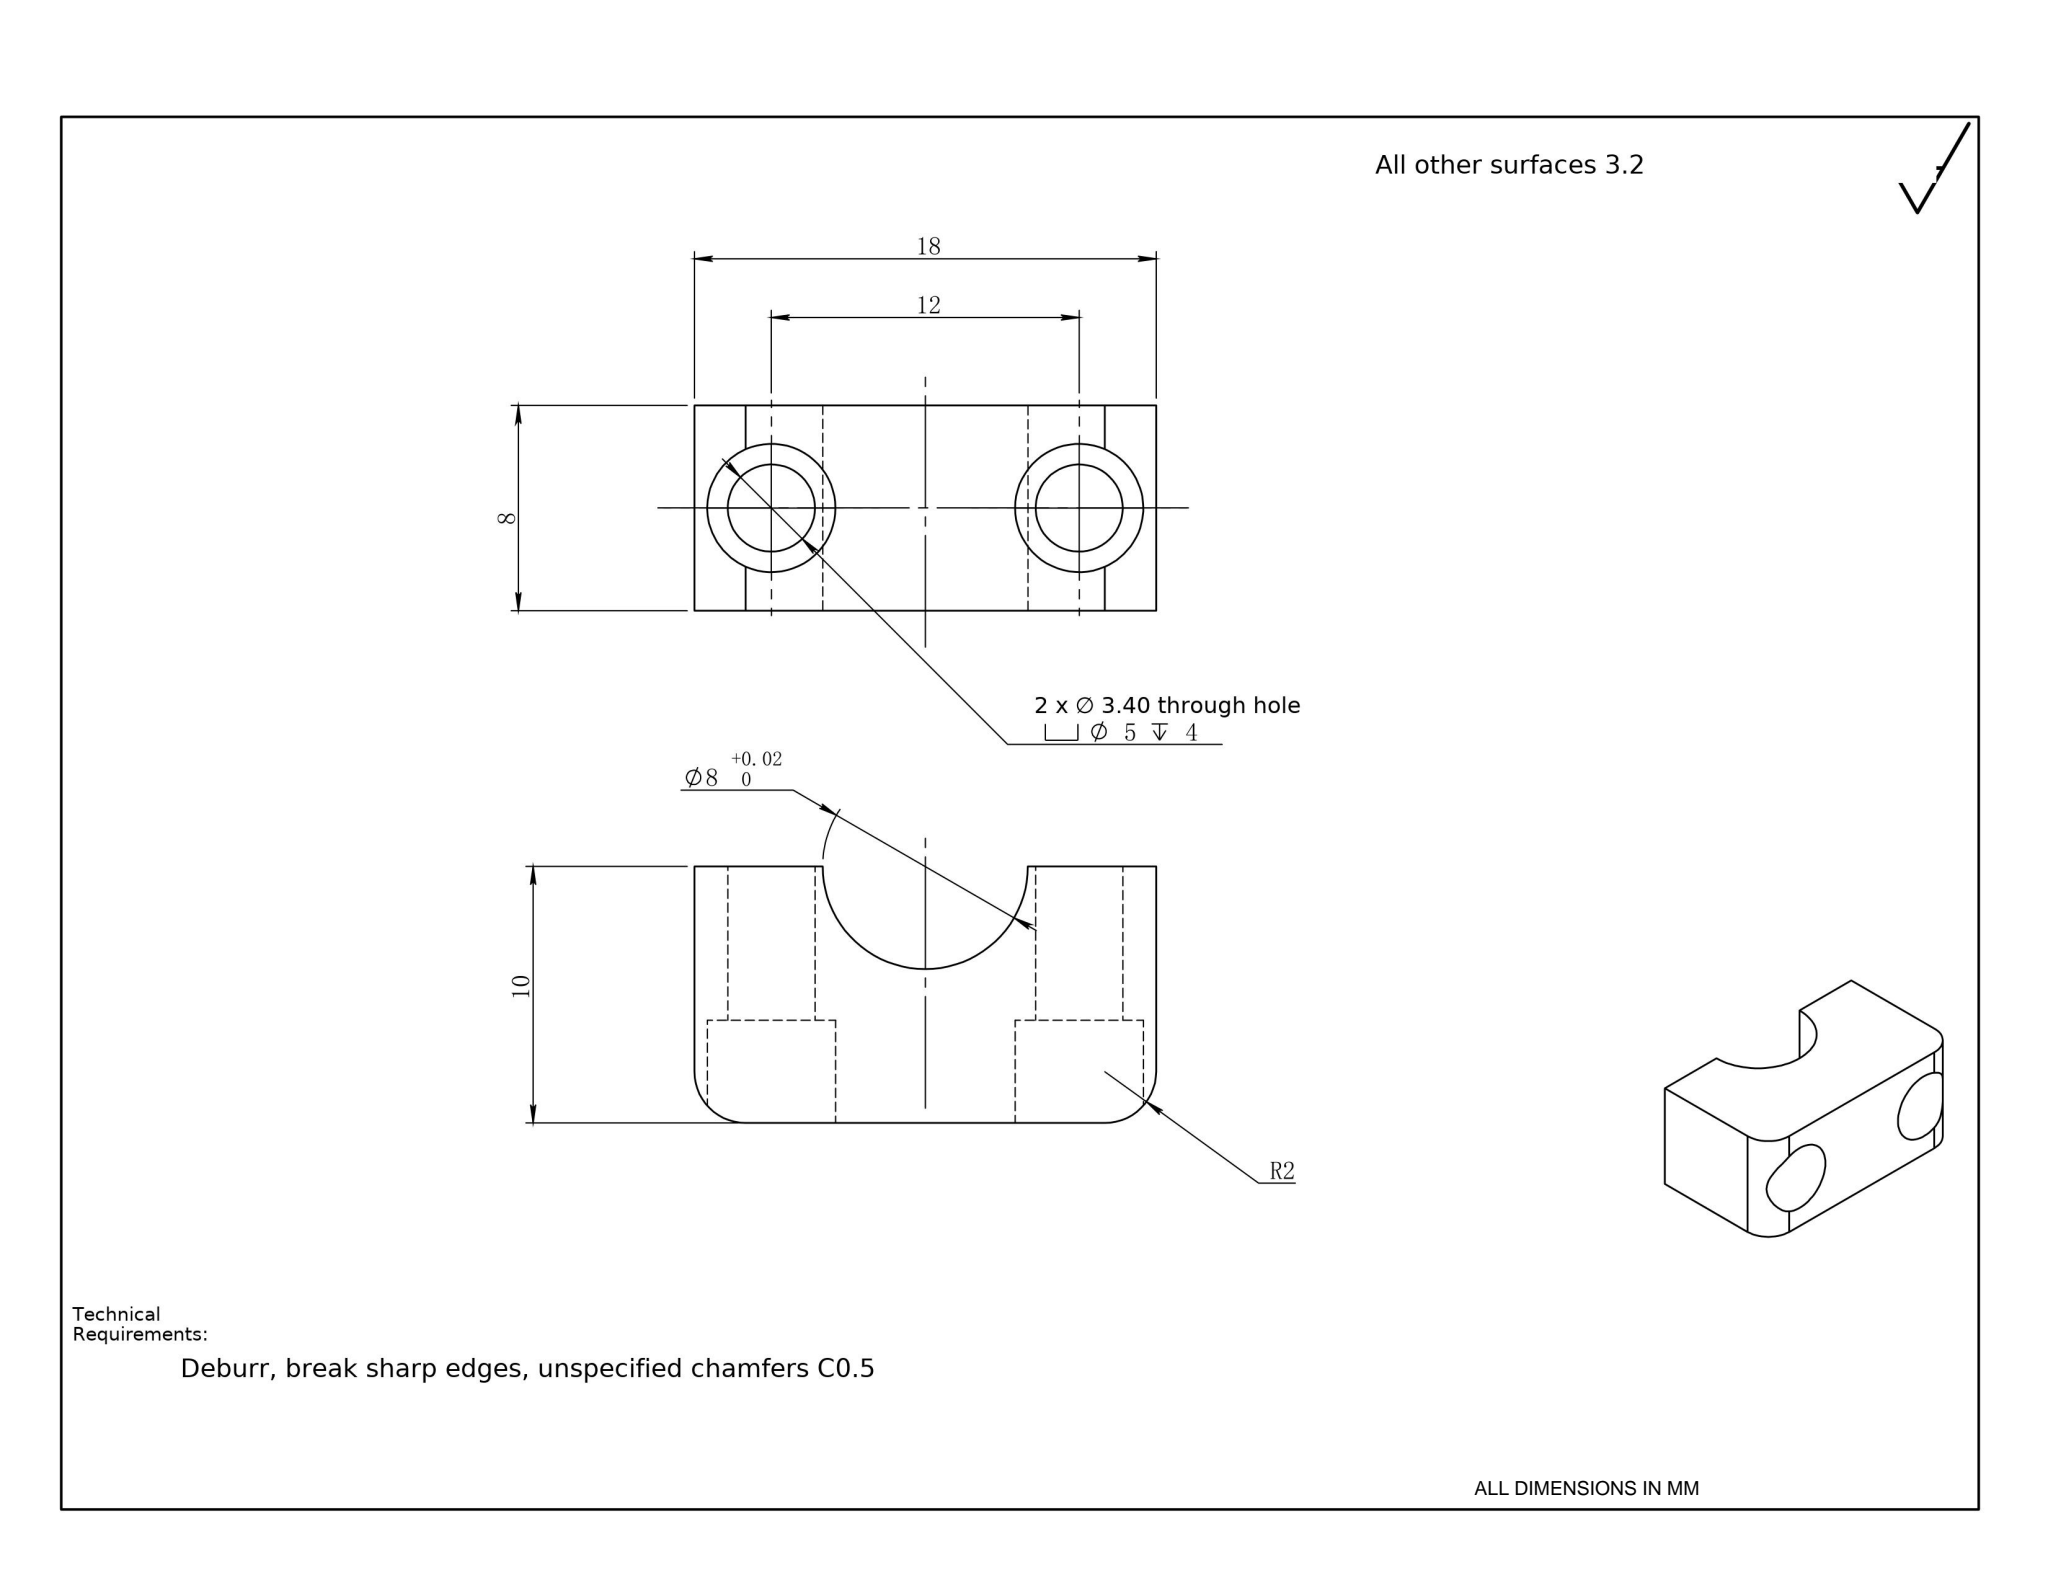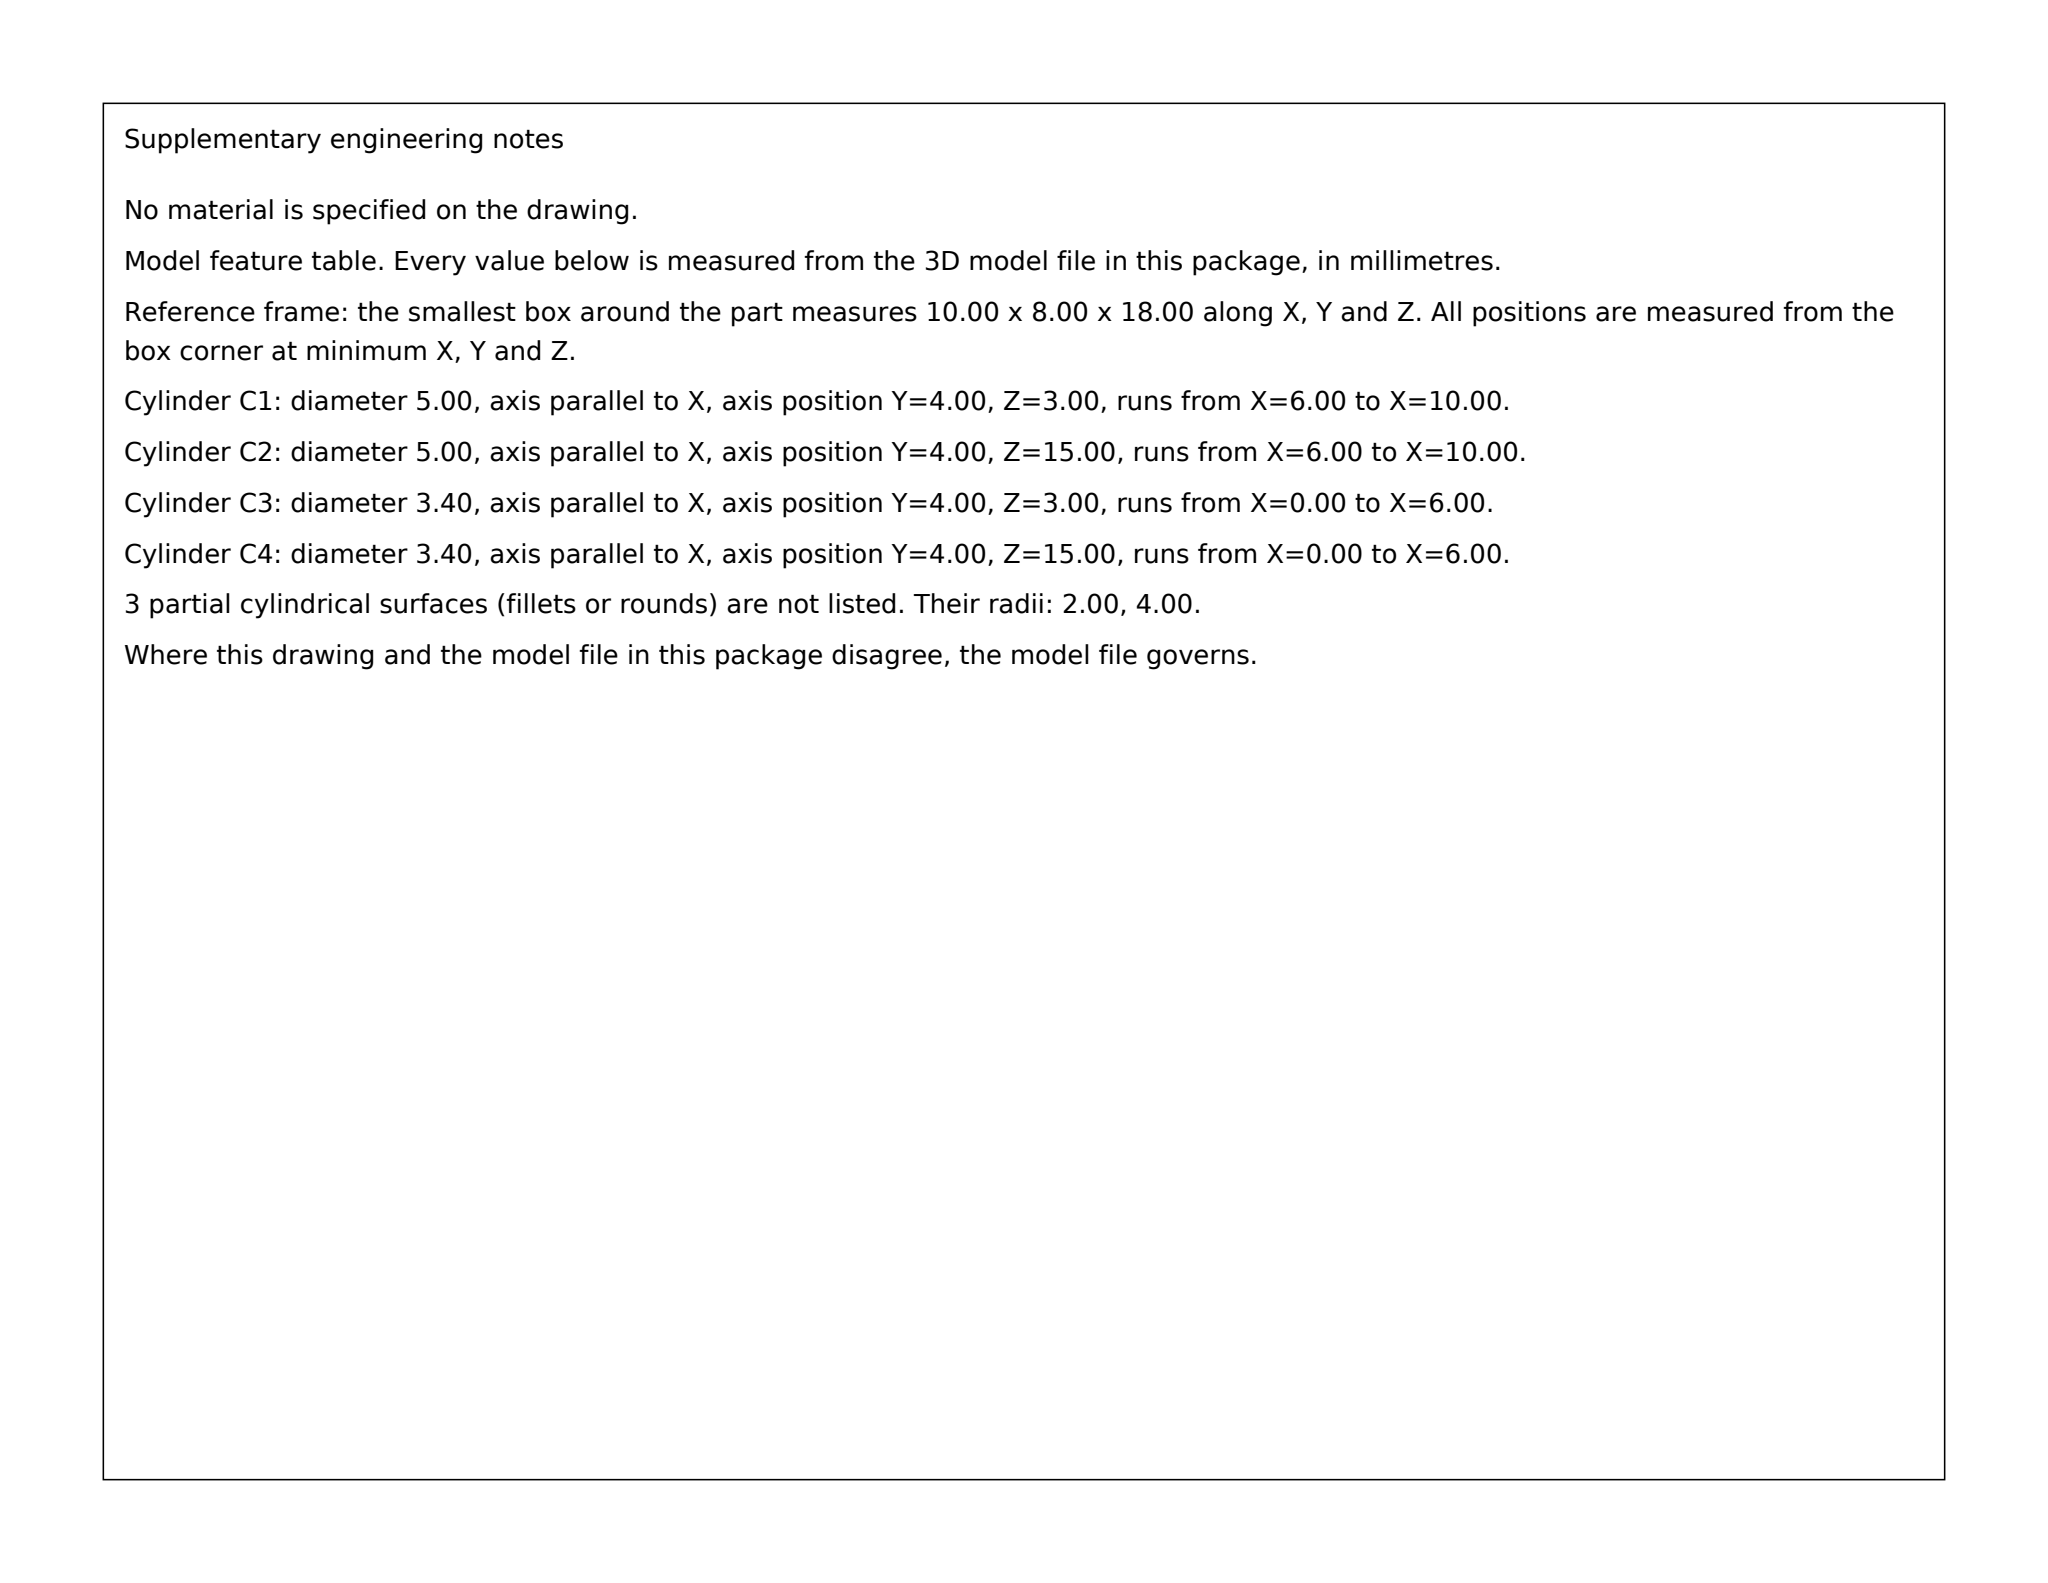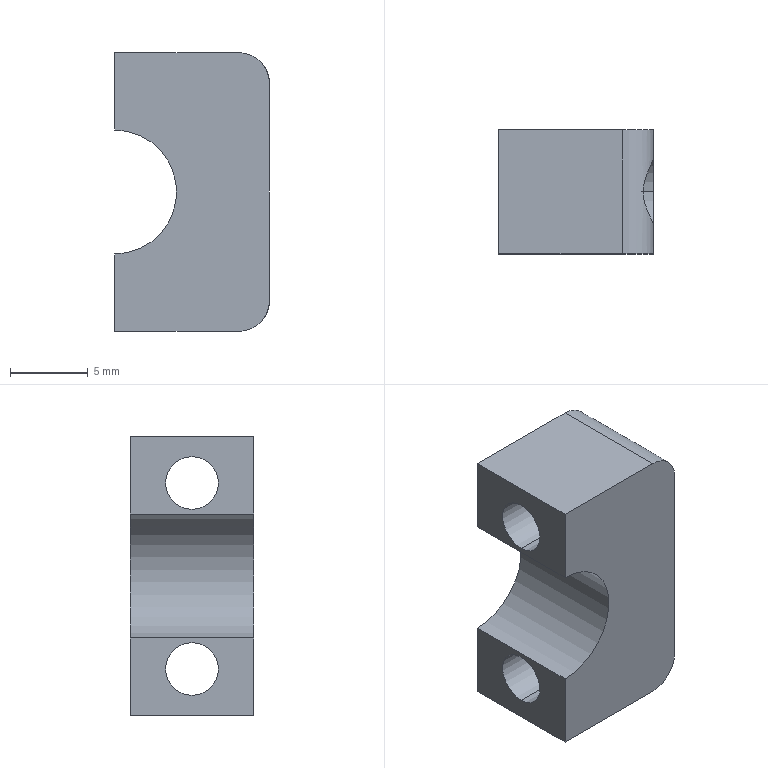Part | SolidWorks | mm | 1 solid | 20 faces | box 10 x 8 x 18 mm | volume 961 mm3 | cylinder 11 | plane 9 | commonest cylinder face diameters 5 x4 3.4 x4 4 x2 8 x1
STEP:
#1=CARTESIAN_POINT('',(1.,0.,8.5));
#2=VERTEX_POINT('',#1);
#3=CARTESIAN_POINT('',(1.,0.,3.5));
#4=VERTEX_POINT('',#3);
#5=CARTESIAN_POINT('',(1.,0.,6.));
#6=DIRECTION('',(1.,0.,0.));
#7=DIRECTION('',(0.,0.,-1.));
#8=AXIS2_PLACEMENT_3D('',#5,#6,#7);
#9=CIRCLE('',#8,2.5);
#10=EDGE_CURVE('',#2,#4,#9,.T.);
#11=ORIENTED_EDGE('',*,*,#10,.F.);
#12=CARTESIAN_POINT('',(4.323,0.,8.5));
#13=VERTEX_POINT('',#12);
#14=CARTESIAN_POINT('',(5.,0.,8.5));
#15=DIRECTION('',(1.,0.,0.));
#16=VECTOR('',#15,1000.);
#17=LINE('',#14,#16);
#18=EDGE_CURVE('',#2,#13,#17,.T.);
#19=ORIENTED_EDGE('',*,*,#18,.T.);
#20=CARTESIAN_POINT('',(5.,-2.291,7.));
#21=VERTEX_POINT('',#20);
#22=CARTESIAN_POINT('',(4.323,0.,8.5));
#23=CARTESIAN_POINT('',(4.323,-0.126,8.5));
#24=CARTESIAN_POINT('',(4.334,-0.2501,8.49));
#25=CARTESIAN_POINT('',(4.374,-0.4931,8.454));
#26=CARTESIAN_POINT('',(4.403,-0.6133,8.427));
#27=CARTESIAN_POINT('',(4.504,-0.958,8.322));
#28=CARTESIAN_POINT('',(4.591,-1.17,8.222));
#29=CARTESIAN_POINT('',(4.759,-1.565,7.964));
#30=CARTESIAN_POINT('',(4.839,-1.742,7.81));
#31=CARTESIAN_POINT('',(4.961,-2.058,7.44));
#32=CARTESIAN_POINT('',(5.,-2.19,7.231));
#33=CARTESIAN_POINT('',(5.,-2.291,7.));
#34=B_SPLINE_CURVE_WITH_KNOTS('',3,(#22,#23,#24,#25,#26,#27,#28,#29,#30,#31,#32,#33),.UNSPECIFIED.,.F.,.F.,(4,2,2,2,2,4),(0.002976,0.003348,0.00372,0.004464,0.005207,0.005951),.UNSPECIFIED.);
#35=EDGE_CURVE('',#13,#21,#34,.T.);
#36=ORIENTED_EDGE('',*,*,#35,.T.);
#37=CARTESIAN_POINT('',(5.,0.,3.5));
#38=VERTEX_POINT('',#37);
#39=CARTESIAN_POINT('',(5.,0.,6.));
#40=DIRECTION('',(1.,0.,0.));
#41=DIRECTION('',(0.,0.,-1.));
#42=AXIS2_PLACEMENT_3D('',#39,#40,#41);
#43=CIRCLE('',#42,2.5);
#44=EDGE_CURVE('',#21,#38,#43,.T.);
#45=ORIENTED_EDGE('',*,*,#44,.T.);
#46=CARTESIAN_POINT('',(5.,0.,3.5));
#47=DIRECTION('',(1.,0.,0.));
#48=VECTOR('',#47,1000.);
#49=LINE('',#46,#48);
#50=EDGE_CURVE('',#4,#38,#49,.T.);
#51=ORIENTED_EDGE('',*,*,#50,.F.);
#52=EDGE_LOOP('',(#11,#19,#36,#45,#51));
#53=FACE_OUTER_BOUND('',#52,.T.);
#54=CARTESIAN_POINT('',(5.,0.,6.));
#55=DIRECTION('',(1.,0.,0.));
#56=DIRECTION('',(0.,0.,-1.));
#57=AXIS2_PLACEMENT_3D('',#54,#55,#56);
#58=CYLINDRICAL_SURFACE('',#57,2.5);
#59=ADVANCED_FACE('',(#53),#58,.F.);
#60=CARTESIAN_POINT('',(-5.,0.,7.7));
#61=VERTEX_POINT('',#60);
#62=CARTESIAN_POINT('',(-5.,0.,4.3));
#63=VERTEX_POINT('',#62);
#64=CARTESIAN_POINT('',(-5.,0.,6.));
#65=DIRECTION('',(1.,0.,0.));
#66=DIRECTION('',(0.,0.,-1.));
#67=AXIS2_PLACEMENT_3D('',#64,#65,#66);
#68=CIRCLE('',#67,1.7);
#69=EDGE_CURVE('',#61,#63,#68,.T.);
#70=ORIENTED_EDGE('',*,*,#69,.F.);
#71=CARTESIAN_POINT('',(1.,0.,7.7));
#72=VERTEX_POINT('',#71);
#73=CARTESIAN_POINT('',(5.,0.,7.7));
#74=DIRECTION('',(1.,0.,0.));
#75=VECTOR('',#74,1000.);
#76=LINE('',#73,#75);
#77=EDGE_CURVE('',#61,#72,#76,.T.);
#78=ORIENTED_EDGE('',*,*,#77,.T.);
#79=CARTESIAN_POINT('',(1.,0.,4.3));
#80=VERTEX_POINT('',#79);
#81=CARTESIAN_POINT('',(1.,0.,6.));
#82=DIRECTION('',(1.,0.,0.));
#83=DIRECTION('',(0.,0.,-1.));
#84=AXIS2_PLACEMENT_3D('',#81,#82,#83);
#85=CIRCLE('',#84,1.7);
#86=EDGE_CURVE('',#72,#80,#85,.T.);
#87=ORIENTED_EDGE('',*,*,#86,.T.);
#88=CARTESIAN_POINT('',(5.,0.,4.3));
#89=DIRECTION('',(1.,0.,0.));
#90=VECTOR('',#89,1000.);
#91=LINE('',#88,#90);
#92=EDGE_CURVE('',#63,#80,#91,.T.);
#93=ORIENTED_EDGE('',*,*,#92,.F.);
#94=EDGE_LOOP('',(#70,#78,#87,#93));
#95=FACE_OUTER_BOUND('',#94,.T.);
#96=CARTESIAN_POINT('',(5.,0.,6.));
#97=DIRECTION('',(1.,0.,0.));
#98=DIRECTION('',(0.,0.,-1.));
#99=AXIS2_PLACEMENT_3D('',#96,#97,#98);
#100=CYLINDRICAL_SURFACE('',#99,1.7);
#101=ADVANCED_FACE('',(#95),#100,.F.);
#102=CARTESIAN_POINT('',(1.,0.,-3.5));
#103=VERTEX_POINT('',#102);
#104=CARTESIAN_POINT('',(1.,0.,-8.5));
#105=VERTEX_POINT('',#104);
#106=CARTESIAN_POINT('',(1.,0.,-6.));
#107=DIRECTION('',(1.,0.,0.));
#108=DIRECTION('',(0.,0.,-1.));
#109=AXIS2_PLACEMENT_3D('',#106,#107,#108);
#110=CIRCLE('',#109,2.5);
#111=EDGE_CURVE('',#103,#105,#110,.T.);
#112=ORIENTED_EDGE('',*,*,#111,.F.);
#113=CARTESIAN_POINT('',(5.,0.,-3.5));
#114=VERTEX_POINT('',#113);
#115=CARTESIAN_POINT('',(5.,0.,-3.5));
#116=DIRECTION('',(1.,0.,0.));
#117=VECTOR('',#116,1000.);
#118=LINE('',#115,#117);
#119=EDGE_CURVE('',#103,#114,#118,.T.);
#120=ORIENTED_EDGE('',*,*,#119,.T.);
#121=CARTESIAN_POINT('',(5.,-2.291,-7.));
#122=VERTEX_POINT('',#121);
#123=CARTESIAN_POINT('',(5.,0.,-6.));
#124=DIRECTION('',(1.,0.,0.));
#125=DIRECTION('',(0.,0.,-1.));
#126=AXIS2_PLACEMENT_3D('',#123,#124,#125);
#127=CIRCLE('',#126,2.5);
#128=EDGE_CURVE('',#114,#122,#127,.T.);
#129=ORIENTED_EDGE('',*,*,#128,.T.);
#130=CARTESIAN_POINT('',(4.323,-0.,-8.5));
#131=VERTEX_POINT('',#130);
#132=CARTESIAN_POINT('',(5.,-2.291,-7.));
#133=CARTESIAN_POINT('',(5.,-2.19,-7.231));
#134=CARTESIAN_POINT('',(4.961,-2.058,-7.44));
#135=CARTESIAN_POINT('',(4.839,-1.742,-7.81));
#136=CARTESIAN_POINT('',(4.759,-1.565,-7.964));
#137=CARTESIAN_POINT('',(4.591,-1.17,-8.222));
#138=CARTESIAN_POINT('',(4.504,-0.9577,-8.322));
#139=CARTESIAN_POINT('',(4.403,-0.6135,-8.427));
#140=CARTESIAN_POINT('',(4.374,-0.493,-8.454));
#141=CARTESIAN_POINT('',(4.334,-0.2498,-8.491));
#142=CARTESIAN_POINT('',(4.323,-0.1261,-8.5));
#143=CARTESIAN_POINT('',(4.323,-0.,-8.5));
#144=B_SPLINE_CURVE_WITH_KNOTS('',3,(#132,#133,#134,#135,#136,#137,#138,#139,#140,#141,#142,#143),.UNSPECIFIED.,.F.,.F.,(4,2,2,2,2,4),(0.,0.0007441,0.001488,0.002232,0.002604,0.002976),.UNSPECIFIED.);
#145=EDGE_CURVE('',#122,#131,#144,.T.);
#146=ORIENTED_EDGE('',*,*,#145,.T.);
#147=CARTESIAN_POINT('',(5.,0.,-8.5));
#148=DIRECTION('',(1.,0.,0.));
#149=VECTOR('',#148,1000.);
#150=LINE('',#147,#149);
#151=EDGE_CURVE('',#105,#131,#150,.T.);
#152=ORIENTED_EDGE('',*,*,#151,.F.);
#153=EDGE_LOOP('',(#112,#120,#129,#146,#152));
#154=FACE_OUTER_BOUND('',#153,.T.);
#155=CARTESIAN_POINT('',(5.,0.,-6.));
#156=DIRECTION('',(1.,0.,0.));
#157=DIRECTION('',(0.,0.,-1.));
#158=AXIS2_PLACEMENT_3D('',#155,#156,#157);
#159=CYLINDRICAL_SURFACE('',#158,2.5);
#160=ADVANCED_FACE('',(#154),#159,.F.);
#161=CARTESIAN_POINT('',(-5.,0.,-4.3));
#162=VERTEX_POINT('',#161);
#163=CARTESIAN_POINT('',(-5.,0.,-7.7));
#164=VERTEX_POINT('',#163);
#165=CARTESIAN_POINT('',(-5.,0.,-6.));
#166=DIRECTION('',(1.,0.,0.));
#167=DIRECTION('',(0.,0.,-1.));
#168=AXIS2_PLACEMENT_3D('',#165,#166,#167);
#169=CIRCLE('',#168,1.7);
#170=EDGE_CURVE('',#162,#164,#169,.T.);
#171=ORIENTED_EDGE('',*,*,#170,.F.);
#172=CARTESIAN_POINT('',(1.,0.,-4.3));
#173=VERTEX_POINT('',#172);
#174=CARTESIAN_POINT('',(5.,0.,-4.3));
#175=DIRECTION('',(1.,0.,0.));
#176=VECTOR('',#175,1000.);
#177=LINE('',#174,#176);
#178=EDGE_CURVE('',#162,#173,#177,.T.);
#179=ORIENTED_EDGE('',*,*,#178,.T.);
#180=CARTESIAN_POINT('',(1.,0.,-7.7));
#181=VERTEX_POINT('',#180);
#182=CARTESIAN_POINT('',(1.,0.,-6.));
#183=DIRECTION('',(1.,0.,0.));
#184=DIRECTION('',(0.,0.,-1.));
#185=AXIS2_PLACEMENT_3D('',#182,#183,#184);
#186=CIRCLE('',#185,1.7);
#187=EDGE_CURVE('',#173,#181,#186,.T.);
#188=ORIENTED_EDGE('',*,*,#187,.T.);
#189=CARTESIAN_POINT('',(5.,0.,-7.7));
#190=DIRECTION('',(1.,0.,0.));
#191=VECTOR('',#190,1000.);
#192=LINE('',#189,#191);
#193=EDGE_CURVE('',#164,#181,#192,.T.);
#194=ORIENTED_EDGE('',*,*,#193,.F.);
#195=EDGE_LOOP('',(#171,#179,#188,#194));
#196=FACE_OUTER_BOUND('',#195,.T.);
#197=CARTESIAN_POINT('',(5.,0.,-6.));
#198=DIRECTION('',(1.,0.,0.));
#199=DIRECTION('',(0.,0.,-1.));
#200=AXIS2_PLACEMENT_3D('',#197,#198,#199);
#201=CYLINDRICAL_SURFACE('',#200,1.7);
#202=ADVANCED_FACE('',(#196),#201,.F.);
#203=CARTESIAN_POINT('',(-5.,0.,-6.));
#204=DIRECTION('',(1.,0.,0.));
#205=DIRECTION('',(0.,0.,-1.));
#206=AXIS2_PLACEMENT_3D('',#203,#204,#205);
#207=CIRCLE('',#206,1.7);
#208=EDGE_CURVE('',#164,#162,#207,.T.);
#209=ORIENTED_EDGE('',*,*,#208,.T.);
#210=ORIENTED_EDGE('',*,*,#170,.T.);
#211=EDGE_LOOP('',(#209,#210));
#212=FACE_BOUND('',#211,.T.);
#213=CARTESIAN_POINT('',(-5.,-4.,-9.));
#214=VERTEX_POINT('',#213);
#215=CARTESIAN_POINT('',(-5.,-4.,-4.));
#216=VERTEX_POINT('',#215);
#217=CARTESIAN_POINT('',(-5.,-4.,9.));
#218=DIRECTION('',(0.,0.,1.));
#219=VECTOR('',#218,1000.);
#220=LINE('',#217,#219);
#221=EDGE_CURVE('',#214,#216,#220,.T.);
#222=ORIENTED_EDGE('',*,*,#221,.T.);
#223=CARTESIAN_POINT('',(-5.,4.,-4.));
#224=VERTEX_POINT('',#223);
#225=CARTESIAN_POINT('',(-5.,-4.,-4.));
#226=DIRECTION('',(0.,1.,0.));
#227=VECTOR('',#226,1000.);
#228=LINE('',#225,#227);
#229=EDGE_CURVE('',#216,#224,#228,.T.);
#230=ORIENTED_EDGE('',*,*,#229,.T.);
#231=CARTESIAN_POINT('',(-5.,4.,-9.));
#232=VERTEX_POINT('',#231);
#233=CARTESIAN_POINT('',(-5.,4.,9.));
#234=DIRECTION('',(0.,0.,1.));
#235=VECTOR('',#234,1000.);
#236=LINE('',#233,#235);
#237=EDGE_CURVE('',#232,#224,#236,.T.);
#238=ORIENTED_EDGE('',*,*,#237,.F.);
#239=CARTESIAN_POINT('',(-5.,4.,-9.));
#240=DIRECTION('',(0.,-1.,0.));
#241=VECTOR('',#240,1000.);
#242=LINE('',#239,#241);
#243=EDGE_CURVE('',#232,#214,#242,.T.);
#244=ORIENTED_EDGE('',*,*,#243,.T.);
#245=EDGE_LOOP('',(#222,#230,#238,#244));
#246=FACE_OUTER_BOUND('',#245,.T.);
#247=CARTESIAN_POINT('',(-5.,4.,9.));
#248=DIRECTION('',(1.,0.,0.));
#249=DIRECTION('',(0.,0.,-1.));
#250=AXIS2_PLACEMENT_3D('',#247,#248,#249);
#251=PLANE('',#250);
#252=ADVANCED_FACE('',(#212,#246),#251,.F.);
#253=CARTESIAN_POINT('',(5.,-4.,7.));
#254=VERTEX_POINT('',#253);
#255=CARTESIAN_POINT('',(5.,-4.,-7.));
#256=VERTEX_POINT('',#255);
#257=CARTESIAN_POINT('',(5.,-4.,9.));
#258=DIRECTION('',(0.,0.,-1.));
#259=VECTOR('',#258,1000.);
#260=LINE('',#257,#259);
#261=EDGE_CURVE('',#254,#256,#260,.T.);
#262=ORIENTED_EDGE('',*,*,#261,.T.);
#263=CARTESIAN_POINT('',(5.,4.,-7.));
#264=DIRECTION('',(0.,1.,0.));
#265=VECTOR('',#264,1000.);
#266=LINE('',#263,#265);
#267=EDGE_CURVE('',#256,#122,#266,.T.);
#268=ORIENTED_EDGE('',*,*,#267,.T.);
#269=ORIENTED_EDGE('',*,*,#128,.F.);
#270=CARTESIAN_POINT('',(5.,2.291,-7.));
#271=VERTEX_POINT('',#270);
#272=CARTESIAN_POINT('',(5.,0.,-6.));
#273=DIRECTION('',(1.,0.,0.));
#274=DIRECTION('',(0.,0.,-1.));
#275=AXIS2_PLACEMENT_3D('',#272,#273,#274);
#276=CIRCLE('',#275,2.5);
#277=EDGE_CURVE('',#271,#114,#276,.T.);
#278=ORIENTED_EDGE('',*,*,#277,.F.);
#279=CARTESIAN_POINT('',(5.,4.,-7.));
#280=VERTEX_POINT('',#279);
#281=CARTESIAN_POINT('',(5.,4.,-7.));
#282=DIRECTION('',(0.,1.,0.));
#283=VECTOR('',#282,1000.);
#284=LINE('',#281,#283);
#285=EDGE_CURVE('',#271,#280,#284,.T.);
#286=ORIENTED_EDGE('',*,*,#285,.T.);
#287=CARTESIAN_POINT('',(5.,4.,7.));
#288=VERTEX_POINT('',#287);
#289=CARTESIAN_POINT('',(5.,4.,9.));
#290=DIRECTION('',(0.,0.,-1.));
#291=VECTOR('',#290,1000.);
#292=LINE('',#289,#291);
#293=EDGE_CURVE('',#288,#280,#292,.T.);
#294=ORIENTED_EDGE('',*,*,#293,.F.);
#295=CARTESIAN_POINT('',(5.,2.291,7.));
#296=VERTEX_POINT('',#295);
#297=CARTESIAN_POINT('',(5.,4.,7.));
#298=DIRECTION('',(0.,-1.,0.));
#299=VECTOR('',#298,1000.);
#300=LINE('',#297,#299);
#301=EDGE_CURVE('',#288,#296,#300,.T.);
#302=ORIENTED_EDGE('',*,*,#301,.T.);
#303=CARTESIAN_POINT('',(5.,0.,6.));
#304=DIRECTION('',(1.,0.,0.));
#305=DIRECTION('',(0.,0.,-1.));
#306=AXIS2_PLACEMENT_3D('',#303,#304,#305);
#307=CIRCLE('',#306,2.5);
#308=EDGE_CURVE('',#38,#296,#307,.T.);
#309=ORIENTED_EDGE('',*,*,#308,.F.);
#310=ORIENTED_EDGE('',*,*,#44,.F.);
#311=CARTESIAN_POINT('',(5.,4.,7.));
#312=DIRECTION('',(0.,-1.,0.));
#313=VECTOR('',#312,1000.);
#314=LINE('',#311,#313);
#315=EDGE_CURVE('',#21,#254,#314,.T.);
#316=ORIENTED_EDGE('',*,*,#315,.T.);
#317=EDGE_LOOP('',(#262,#268,#269,#278,#286,#294,#302,#309,#310,#316));
#318=FACE_OUTER_BOUND('',#317,.T.);
#319=CARTESIAN_POINT('',(5.,4.,9.));
#320=DIRECTION('',(-1.,0.,0.));
#321=DIRECTION('',(0.,0.,1.));
#322=AXIS2_PLACEMENT_3D('',#319,#320,#321);
#323=PLANE('',#322);
#324=ADVANCED_FACE('',(#318),#323,.F.);
#325=CARTESIAN_POINT('',(3.,4.,-9.));
#326=VERTEX_POINT('',#325);
#327=CARTESIAN_POINT('',(-5.,4.,-9.));
#328=DIRECTION('',(-1.,0.,0.));
#329=VECTOR('',#328,1000.);
#330=LINE('',#327,#329);
#331=EDGE_CURVE('',#326,#232,#330,.T.);
#332=ORIENTED_EDGE('',*,*,#331,.F.);
#333=CARTESIAN_POINT('',(3.,-4.,-9.));
#334=VERTEX_POINT('',#333);
#335=CARTESIAN_POINT('',(3.,4.,-9.));
#336=DIRECTION('',(0.,-1.,0.));
#337=VECTOR('',#336,1000.);
#338=LINE('',#335,#337);
#339=EDGE_CURVE('',#326,#334,#338,.T.);
#340=ORIENTED_EDGE('',*,*,#339,.T.);
#341=CARTESIAN_POINT('',(-5.,-4.,-9.));
#342=DIRECTION('',(-1.,0.,0.));
#343=VECTOR('',#342,1000.);
#344=LINE('',#341,#343);
#345=EDGE_CURVE('',#334,#214,#344,.T.);
#346=ORIENTED_EDGE('',*,*,#345,.T.);
#347=ORIENTED_EDGE('',*,*,#243,.F.);
#348=EDGE_LOOP('',(#332,#340,#346,#347));
#349=FACE_OUTER_BOUND('',#348,.T.);
#350=CARTESIAN_POINT('',(-5.,4.,-9.));
#351=DIRECTION('',(0.,0.,1.));
#352=DIRECTION('',(1.,0.,0.));
#353=AXIS2_PLACEMENT_3D('',#350,#351,#352);
#354=PLANE('',#353);
#355=ADVANCED_FACE('',(#349),#354,.F.);
#356=CARTESIAN_POINT('',(-5.,0.,6.));
#357=DIRECTION('',(1.,0.,0.));
#358=DIRECTION('',(0.,0.,-1.));
#359=AXIS2_PLACEMENT_3D('',#356,#357,#358);
#360=CIRCLE('',#359,1.7);
#361=EDGE_CURVE('',#63,#61,#360,.T.);
#362=ORIENTED_EDGE('',*,*,#361,.T.);
#363=ORIENTED_EDGE('',*,*,#69,.T.);
#364=EDGE_LOOP('',(#362,#363));
#365=FACE_BOUND('',#364,.T.);
#366=CARTESIAN_POINT('',(-5.,4.,4.));
#367=VERTEX_POINT('',#366);
#368=CARTESIAN_POINT('',(-5.,4.,9.));
#369=VERTEX_POINT('',#368);
#370=CARTESIAN_POINT('',(-5.,4.,9.));
#371=DIRECTION('',(0.,0.,1.));
#372=VECTOR('',#371,1000.);
#373=LINE('',#370,#372);
#374=EDGE_CURVE('',#367,#369,#373,.T.);
#375=ORIENTED_EDGE('',*,*,#374,.F.);
#376=CARTESIAN_POINT('',(-5.,-4.,4.));
#377=VERTEX_POINT('',#376);
#378=CARTESIAN_POINT('',(-5.,-4.,4.));
#379=DIRECTION('',(0.,-1.,0.));
#380=VECTOR('',#379,1000.);
#381=LINE('',#378,#380);
#382=EDGE_CURVE('',#367,#377,#381,.T.);
#383=ORIENTED_EDGE('',*,*,#382,.T.);
#384=CARTESIAN_POINT('',(-5.,-4.,9.));
#385=VERTEX_POINT('',#384);
#386=CARTESIAN_POINT('',(-5.,-4.,9.));
#387=DIRECTION('',(0.,0.,1.));
#388=VECTOR('',#387,1000.);
#389=LINE('',#386,#388);
#390=EDGE_CURVE('',#377,#385,#389,.T.);
#391=ORIENTED_EDGE('',*,*,#390,.T.);
#392=CARTESIAN_POINT('',(-5.,4.,9.));
#393=DIRECTION('',(0.,-1.,0.));
#394=VECTOR('',#393,1000.);
#395=LINE('',#392,#394);
#396=EDGE_CURVE('',#369,#385,#395,.T.);
#397=ORIENTED_EDGE('',*,*,#396,.F.);
#398=EDGE_LOOP('',(#375,#383,#391,#397));
#399=FACE_OUTER_BOUND('',#398,.T.);
#400=CARTESIAN_POINT('',(-5.,4.,9.));
#401=DIRECTION('',(1.,0.,0.));
#402=DIRECTION('',(0.,0.,-1.));
#403=AXIS2_PLACEMENT_3D('',#400,#401,#402);
#404=PLANE('',#403);
#405=ADVANCED_FACE('',(#365,#399),#404,.F.);
#406=CARTESIAN_POINT('',(3.,-4.,9.));
#407=VERTEX_POINT('',#406);
#408=CARTESIAN_POINT('',(-5.,-4.,9.));
#409=DIRECTION('',(1.,0.,0.));
#410=VECTOR('',#409,1000.);
#411=LINE('',#408,#410);
#412=EDGE_CURVE('',#385,#407,#411,.T.);
#413=ORIENTED_EDGE('',*,*,#412,.T.);
#414=CARTESIAN_POINT('',(3.,4.,9.));
#415=VERTEX_POINT('',#414);
#416=CARTESIAN_POINT('',(3.,4.,9.));
#417=DIRECTION('',(0.,1.,0.));
#418=VECTOR('',#417,1000.);
#419=LINE('',#416,#418);
#420=EDGE_CURVE('',#407,#415,#419,.T.);
#421=ORIENTED_EDGE('',*,*,#420,.T.);
#422=CARTESIAN_POINT('',(-5.,4.,9.));
#423=DIRECTION('',(1.,0.,0.));
#424=VECTOR('',#423,1000.);
#425=LINE('',#422,#424);
#426=EDGE_CURVE('',#369,#415,#425,.T.);
#427=ORIENTED_EDGE('',*,*,#426,.F.);
#428=ORIENTED_EDGE('',*,*,#396,.T.);
#429=EDGE_LOOP('',(#413,#421,#427,#428));
#430=FACE_OUTER_BOUND('',#429,.T.);
#431=CARTESIAN_POINT('',(-5.,4.,9.));
#432=DIRECTION('',(0.,0.,-1.));
#433=DIRECTION('',(-1.,0.,0.));
#434=AXIS2_PLACEMENT_3D('',#431,#432,#433);
#435=PLANE('',#434);
#436=ADVANCED_FACE('',(#430),#435,.F.);
#437=ORIENTED_EDGE('',*,*,#293,.T.);
#438=CARTESIAN_POINT('',(3.,4.,-7.));
#439=DIRECTION('',(0.,1.,0.));
#440=DIRECTION('',(0.,0.,-1.));
#441=AXIS2_PLACEMENT_3D('',#438,#439,#440);
#442=CIRCLE('',#441,2.);
#443=EDGE_CURVE('',#280,#326,#442,.T.);
#444=ORIENTED_EDGE('',*,*,#443,.T.);
#445=ORIENTED_EDGE('',*,*,#331,.T.);
#446=ORIENTED_EDGE('',*,*,#237,.T.);
#447=CARTESIAN_POINT('',(-5.,4.,0.));
#448=DIRECTION('',(0.,1.,0.));
#449=DIRECTION('',(0.,0.,1.));
#450=AXIS2_PLACEMENT_3D('',#447,#448,#449);
#451=CIRCLE('',#450,4.);
#452=EDGE_CURVE('',#367,#224,#451,.T.);
#453=ORIENTED_EDGE('',*,*,#452,.F.);
#454=ORIENTED_EDGE('',*,*,#374,.T.);
#455=ORIENTED_EDGE('',*,*,#426,.T.);
#456=CARTESIAN_POINT('',(3.,4.,7.));
#457=DIRECTION('',(0.,1.,0.));
#458=DIRECTION('',(0.,0.,-1.));
#459=AXIS2_PLACEMENT_3D('',#456,#457,#458);
#460=CIRCLE('',#459,2.);
#461=EDGE_CURVE('',#415,#288,#460,.T.);
#462=ORIENTED_EDGE('',*,*,#461,.T.);
#463=EDGE_LOOP('',(#437,#444,#445,#446,#453,#454,#455,#462));
#464=FACE_OUTER_BOUND('',#463,.T.);
#465=CARTESIAN_POINT('',(0.,4.,0.));
#466=DIRECTION('',(0.,-1.,0.));
#467=DIRECTION('',(0.,0.,-1.));
#468=AXIS2_PLACEMENT_3D('',#465,#466,#467);
#469=PLANE('',#468);
#470=ADVANCED_FACE('',(#464),#469,.F.);
#471=ORIENTED_EDGE('',*,*,#345,.F.);
#472=CARTESIAN_POINT('',(3.,-4.,-7.));
#473=DIRECTION('',(0.,-1.,0.));
#474=DIRECTION('',(0.,0.,-1.));
#475=AXIS2_PLACEMENT_3D('',#472,#473,#474);
#476=CIRCLE('',#475,2.);
#477=EDGE_CURVE('',#334,#256,#476,.T.);
#478=ORIENTED_EDGE('',*,*,#477,.T.);
#479=ORIENTED_EDGE('',*,*,#261,.F.);
#480=CARTESIAN_POINT('',(3.,-4.,7.));
#481=DIRECTION('',(0.,-1.,0.));
#482=DIRECTION('',(0.,0.,-1.));
#483=AXIS2_PLACEMENT_3D('',#480,#481,#482);
#484=CIRCLE('',#483,2.);
#485=EDGE_CURVE('',#254,#407,#484,.T.);
#486=ORIENTED_EDGE('',*,*,#485,.T.);
#487=ORIENTED_EDGE('',*,*,#412,.F.);
#488=ORIENTED_EDGE('',*,*,#390,.F.);
#489=CARTESIAN_POINT('',(-5.,-4.,0.));
#490=DIRECTION('',(0.,1.,0.));
#491=DIRECTION('',(0.,0.,1.));
#492=AXIS2_PLACEMENT_3D('',#489,#490,#491);
#493=CIRCLE('',#492,4.);
#494=EDGE_CURVE('',#377,#216,#493,.T.);
#495=ORIENTED_EDGE('',*,*,#494,.T.);
#496=ORIENTED_EDGE('',*,*,#221,.F.);
#497=EDGE_LOOP('',(#471,#478,#479,#486,#487,#488,#495,#496));
#498=FACE_OUTER_BOUND('',#497,.T.);
#499=CARTESIAN_POINT('',(0.,-4.,0.));
#500=DIRECTION('',(0.,-1.,0.));
#501=DIRECTION('',(0.,0.,-1.));
#502=AXIS2_PLACEMENT_3D('',#499,#500,#501);
#503=PLANE('',#502);
#504=ADVANCED_FACE('',(#498),#503,.T.);
#505=ORIENTED_EDGE('',*,*,#494,.F.);
#506=ORIENTED_EDGE('',*,*,#382,.F.);
#507=ORIENTED_EDGE('',*,*,#452,.T.);
#508=ORIENTED_EDGE('',*,*,#229,.F.);
#509=EDGE_LOOP('',(#505,#506,#507,#508));
#510=FACE_OUTER_BOUND('',#509,.T.);
#511=CARTESIAN_POINT('',(-5.,-4.,0.));
#512=DIRECTION('',(0.,1.,0.));
#513=DIRECTION('',(0.,0.,1.));
#514=AXIS2_PLACEMENT_3D('',#511,#512,#513);
#515=CYLINDRICAL_SURFACE('',#514,4.);
#516=ADVANCED_FACE('',(#510),#515,.F.);
#517=ORIENTED_EDGE('',*,*,#178,.F.);
#518=ORIENTED_EDGE('',*,*,#208,.F.);
#519=ORIENTED_EDGE('',*,*,#193,.T.);
#520=CARTESIAN_POINT('',(1.,0.,-6.));
#521=DIRECTION('',(1.,0.,0.));
#522=DIRECTION('',(0.,0.,-1.));
#523=AXIS2_PLACEMENT_3D('',#520,#521,#522);
#524=CIRCLE('',#523,1.7);
#525=EDGE_CURVE('',#181,#173,#524,.T.);
#526=ORIENTED_EDGE('',*,*,#525,.T.);
#527=EDGE_LOOP('',(#517,#518,#519,#526));
#528=FACE_OUTER_BOUND('',#527,.T.);
#529=CARTESIAN_POINT('',(5.,0.,-6.));
#530=DIRECTION('',(1.,0.,0.));
#531=DIRECTION('',(0.,0.,-1.));
#532=AXIS2_PLACEMENT_3D('',#529,#530,#531);
#533=CYLINDRICAL_SURFACE('',#532,1.7);
#534=ADVANCED_FACE('',(#528),#533,.F.);
#535=ORIENTED_EDGE('',*,*,#525,.F.);
#536=ORIENTED_EDGE('',*,*,#187,.F.);
#537=EDGE_LOOP('',(#535,#536));
#538=FACE_BOUND('',#537,.T.);
#539=CARTESIAN_POINT('',(1.,0.,-6.));
#540=DIRECTION('',(1.,0.,0.));
#541=DIRECTION('',(0.,0.,-1.));
#542=AXIS2_PLACEMENT_3D('',#539,#540,#541);
#543=CIRCLE('',#542,2.5);
#544=EDGE_CURVE('',#105,#103,#543,.T.);
#545=ORIENTED_EDGE('',*,*,#544,.T.);
#546=ORIENTED_EDGE('',*,*,#111,.T.);
#547=EDGE_LOOP('',(#545,#546));
#548=FACE_OUTER_BOUND('',#547,.T.);
#549=CARTESIAN_POINT('',(1.,1.7,-6.));
#550=DIRECTION('',(-1.,0.,0.));
#551=DIRECTION('',(0.,0.,1.));
#552=AXIS2_PLACEMENT_3D('',#549,#550,#551);
#553=PLANE('',#552);
#554=ADVANCED_FACE('',(#538,#548),#553,.F.);
#555=ORIENTED_EDGE('',*,*,#119,.F.);
#556=ORIENTED_EDGE('',*,*,#544,.F.);
#557=ORIENTED_EDGE('',*,*,#151,.T.);
#558=CARTESIAN_POINT('',(4.323,-0.,-8.5));
#559=CARTESIAN_POINT('',(4.323,0.126,-8.5));
#560=CARTESIAN_POINT('',(4.334,0.2501,-8.49));
#561=CARTESIAN_POINT('',(4.374,0.4931,-8.454));
#562=CARTESIAN_POINT('',(4.403,0.6133,-8.427));
#563=CARTESIAN_POINT('',(4.504,0.958,-8.322));
#564=CARTESIAN_POINT('',(4.591,1.17,-8.222));
#565=CARTESIAN_POINT('',(4.759,1.565,-7.964));
#566=CARTESIAN_POINT('',(4.839,1.742,-7.81));
#567=CARTESIAN_POINT('',(4.961,2.058,-7.44));
#568=CARTESIAN_POINT('',(5.,2.19,-7.231));
#569=CARTESIAN_POINT('',(5.,2.291,-7.));
#570=B_SPLINE_CURVE_WITH_KNOTS('',3,(#558,#559,#560,#561,#562,#563,#564,#565,#566,#567,#568,#569),.UNSPECIFIED.,.F.,.F.,(4,2,2,2,2,4),(0.002976,0.003348,0.00372,0.004464,0.005207,0.005951),.UNSPECIFIED.);
#571=EDGE_CURVE('',#131,#271,#570,.T.);
#572=ORIENTED_EDGE('',*,*,#571,.T.);
#573=ORIENTED_EDGE('',*,*,#277,.T.);
#574=EDGE_LOOP('',(#555,#556,#557,#572,#573));
#575=FACE_OUTER_BOUND('',#574,.T.);
#576=CARTESIAN_POINT('',(5.,0.,-6.));
#577=DIRECTION('',(1.,0.,0.));
#578=DIRECTION('',(0.,0.,-1.));
#579=AXIS2_PLACEMENT_3D('',#576,#577,#578);
#580=CYLINDRICAL_SURFACE('',#579,2.5);
#581=ADVANCED_FACE('',(#575),#580,.F.);
#582=ORIENTED_EDGE('',*,*,#77,.F.);
#583=ORIENTED_EDGE('',*,*,#361,.F.);
#584=ORIENTED_EDGE('',*,*,#92,.T.);
#585=CARTESIAN_POINT('',(1.,0.,6.));
#586=DIRECTION('',(1.,0.,0.));
#587=DIRECTION('',(0.,0.,-1.));
#588=AXIS2_PLACEMENT_3D('',#585,#586,#587);
#589=CIRCLE('',#588,1.7);
#590=EDGE_CURVE('',#80,#72,#589,.T.);
#591=ORIENTED_EDGE('',*,*,#590,.T.);
#592=EDGE_LOOP('',(#582,#583,#584,#591));
#593=FACE_OUTER_BOUND('',#592,.T.);
#594=CARTESIAN_POINT('',(5.,0.,6.));
#595=DIRECTION('',(1.,0.,0.));
#596=DIRECTION('',(0.,0.,-1.));
#597=AXIS2_PLACEMENT_3D('',#594,#595,#596);
#598=CYLINDRICAL_SURFACE('',#597,1.7);
#599=ADVANCED_FACE('',(#593),#598,.F.);
#600=ORIENTED_EDGE('',*,*,#590,.F.);
#601=ORIENTED_EDGE('',*,*,#86,.F.);
#602=EDGE_LOOP('',(#600,#601));
#603=FACE_BOUND('',#602,.T.);
#604=CARTESIAN_POINT('',(1.,0.,6.));
#605=DIRECTION('',(1.,0.,0.));
#606=DIRECTION('',(0.,0.,-1.));
#607=AXIS2_PLACEMENT_3D('',#604,#605,#606);
#608=CIRCLE('',#607,2.5);
#609=EDGE_CURVE('',#4,#2,#608,.T.);
#610=ORIENTED_EDGE('',*,*,#609,.T.);
#611=ORIENTED_EDGE('',*,*,#10,.T.);
#612=EDGE_LOOP('',(#610,#611));
#613=FACE_OUTER_BOUND('',#612,.T.);
#614=CARTESIAN_POINT('',(1.,1.7,6.));
#615=DIRECTION('',(-1.,0.,0.));
#616=DIRECTION('',(0.,0.,1.));
#617=AXIS2_PLACEMENT_3D('',#614,#615,#616);
#618=PLANE('',#617);
#619=ADVANCED_FACE('',(#603,#613),#618,.F.);
#620=ORIENTED_EDGE('',*,*,#18,.F.);
#621=ORIENTED_EDGE('',*,*,#609,.F.);
#622=ORIENTED_EDGE('',*,*,#50,.T.);
#623=ORIENTED_EDGE('',*,*,#308,.T.);
#624=CARTESIAN_POINT('',(5.,2.291,7.));
#625=CARTESIAN_POINT('',(5.,2.19,7.231));
#626=CARTESIAN_POINT('',(4.961,2.058,7.44));
#627=CARTESIAN_POINT('',(4.839,1.742,7.81));
#628=CARTESIAN_POINT('',(4.759,1.565,7.964));
#629=CARTESIAN_POINT('',(4.591,1.17,8.222));
#630=CARTESIAN_POINT('',(4.504,0.9577,8.322));
#631=CARTESIAN_POINT('',(4.403,0.6135,8.427));
#632=CARTESIAN_POINT('',(4.374,0.493,8.454));
#633=CARTESIAN_POINT('',(4.334,0.2498,8.491));
#634=CARTESIAN_POINT('',(4.323,0.1261,8.5));
#635=CARTESIAN_POINT('',(4.323,0.,8.5));
#636=B_SPLINE_CURVE_WITH_KNOTS('',3,(#624,#625,#626,#627,#628,#629,#630,#631,#632,#633,#634,#635),.UNSPECIFIED.,.F.,.F.,(4,2,2,2,2,4),(0.,0.0007441,0.001488,0.002232,0.002604,0.002976),.UNSPECIFIED.);
#637=EDGE_CURVE('',#296,#13,#636,.T.);
#638=ORIENTED_EDGE('',*,*,#637,.T.);
#639=EDGE_LOOP('',(#620,#621,#622,#623,#638));
#640=FACE_OUTER_BOUND('',#639,.T.);
#641=CARTESIAN_POINT('',(5.,0.,6.));
#642=DIRECTION('',(1.,0.,0.));
#643=DIRECTION('',(0.,0.,-1.));
#644=AXIS2_PLACEMENT_3D('',#641,#642,#643);
#645=CYLINDRICAL_SURFACE('',#644,2.5);
#646=ADVANCED_FACE('',(#640),#645,.F.);
#647=ORIENTED_EDGE('',*,*,#145,.F.);
#648=ORIENTED_EDGE('',*,*,#267,.F.);
#649=ORIENTED_EDGE('',*,*,#477,.F.);
#650=ORIENTED_EDGE('',*,*,#339,.F.);
#651=ORIENTED_EDGE('',*,*,#443,.F.);
#652=ORIENTED_EDGE('',*,*,#285,.F.);
#653=ORIENTED_EDGE('',*,*,#571,.F.);
#654=EDGE_LOOP('',(#647,#648,#649,#650,#651,#652,#653));
#655=FACE_OUTER_BOUND('',#654,.T.);
#656=CARTESIAN_POINT('',(3.,4.,-7.));
#657=DIRECTION('',(0.,-1.,0.));
#658=DIRECTION('',(0.,0.,-1.));
#659=AXIS2_PLACEMENT_3D('',#656,#657,#658);
#660=CYLINDRICAL_SURFACE('',#659,2.);
#661=ADVANCED_FACE('',(#655),#660,.T.);
#662=ORIENTED_EDGE('',*,*,#461,.F.);
#663=ORIENTED_EDGE('',*,*,#420,.F.);
#664=ORIENTED_EDGE('',*,*,#485,.F.);
#665=ORIENTED_EDGE('',*,*,#315,.F.);
#666=ORIENTED_EDGE('',*,*,#35,.F.);
#667=ORIENTED_EDGE('',*,*,#637,.F.);
#668=ORIENTED_EDGE('',*,*,#301,.F.);
#669=EDGE_LOOP('',(#662,#663,#664,#665,#666,#667,#668));
#670=FACE_OUTER_BOUND('',#669,.T.);
#671=CARTESIAN_POINT('',(3.,4.,7.));
#672=DIRECTION('',(0.,-1.,0.));
#673=DIRECTION('',(0.,0.,-1.));
#674=AXIS2_PLACEMENT_3D('',#671,#672,#673);
#675=CYLINDRICAL_SURFACE('',#674,2.);
#676=ADVANCED_FACE('',(#670),#675,.T.);
#677=CLOSED_SHELL('',(#59,#101,#160,#202,#252,#324,#355,#405,#436,#470,#504,#516,#534,#554,#581,#599,#619,#646,#661,#676));
#678=MANIFOLD_SOLID_BREP('',#677);
#679=CARTESIAN_POINT('',(0.,0.,0.));
#680=DIRECTION('',(0.,0.,1.));
#681=DIRECTION('',(1.,0.,0.));
#682=AXIS2_PLACEMENT_3D('',#679,#680,#681);
#683=(LENGTH_UNIT()NAMED_UNIT(*)SI_UNIT(.MILLI.,.METRE.));
#684=UNCERTAINTY_MEASURE_WITH_UNIT(LENGTH_MEASURE(0.00001),#683,'','');
#685=(NAMED_UNIT(*)PLANE_ANGLE_UNIT()SI_UNIT($,.RADIAN.));
#686=(NAMED_UNIT(*)SI_UNIT($,.STERADIAN.)SOLID_ANGLE_UNIT());
#687=(GEOMETRIC_REPRESENTATION_CONTEXT(3)GLOBAL_UNCERTAINTY_ASSIGNED_CONTEXT((#684))GLOBAL_UNIT_ASSIGNED_CONTEXT((#683,#685,#686))REPRESENTATION_CONTEXT('',''));
#688=ADVANCED_BREP_SHAPE_REPRESENTATION('',(#678,#682),#687);